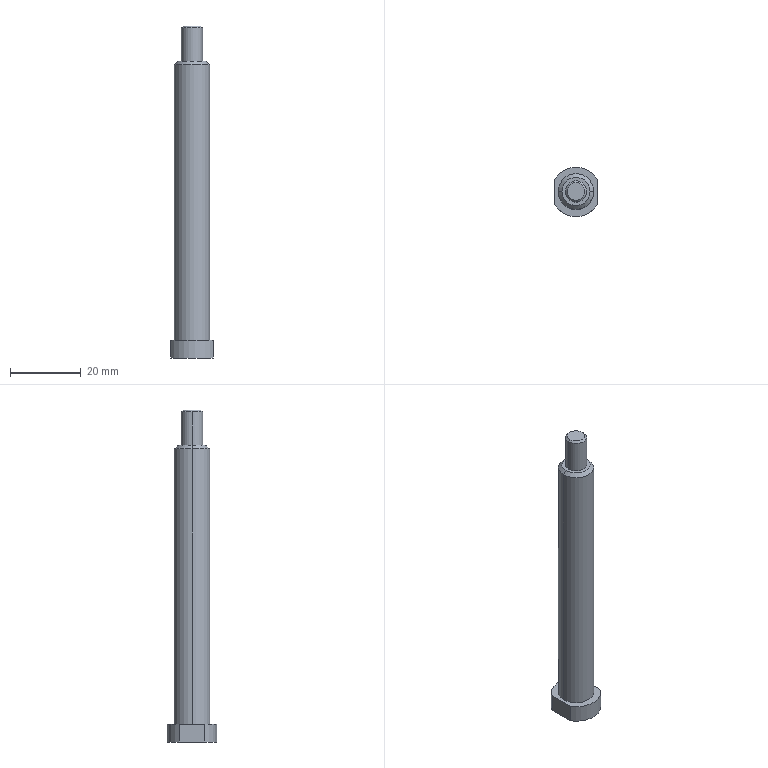Component | SolidWorks | ZTDJ-L-400-04-21-MaterialPortBagClamp-Axis5-2 | 1 solid | 16 faces | box 12 x 14 x 94 mm | volume 7191 mm3 | cylinder 6 | plane 6 | cone 4 | commonest cylinder face diameters 6 x2 10 x2 14 x2 | material 1023 Carbon Steel Sheet (SS)
STEP:
#1=COLOUR_RGB('',0.7922,0.8196,0.9333);
#2=FILL_AREA_STYLE_COLOUR('',#1);
#3=FILL_AREA_STYLE('',(#2));
#4=SURFACE_STYLE_FILL_AREA(#3);
#5=SURFACE_SIDE_STYLE('',(#4));
#6=SURFACE_STYLE_USAGE(.BOTH.,#5);
#7=PRESENTATION_STYLE_ASSIGNMENT((#6));
#8=CARTESIAN_POINT('',(-3.383,-3.314,13.346));
#9=VERTEX_POINT('',#8);
#10=CARTESIAN_POINT('',(-3.58,-3.314,13.346));
#11=VERTEX_POINT('',#10);
#12=CARTESIAN_POINT('',(-3.482,-3.314,13.346));
#13=DIRECTION('',(0.,0.,1.));
#14=DIRECTION('',(1.,0.,0.));
#15=AXIS2_PLACEMENT_3D('',#12,#13,#14);
#16=CIRCLE('',#15,0.09843);
#17=EDGE_CURVE('',#9,#11,#16,.T.);
#18=ORIENTED_EDGE('',*,*,#17,.F.);
#19=CARTESIAN_POINT('',(-3.364,-3.314,13.327));
#20=VERTEX_POINT('',#19);
#21=CARTESIAN_POINT('',(-3.383,-3.314,13.346));
#22=DIRECTION('',(0.7071,0.,-0.7071));
#23=VECTOR('',#22,39.37);
#24=LINE('',#21,#23);
#25=EDGE_CURVE('',#9,#20,#24,.T.);
#26=ORIENTED_EDGE('',*,*,#25,.T.);
#27=CARTESIAN_POINT('',(-3.6,-3.314,13.327));
#28=VERTEX_POINT('',#27);
#29=CARTESIAN_POINT('',(-3.482,-3.314,13.327));
#30=DIRECTION('',(0.,0.,-1.));
#31=DIRECTION('',(1.,0.,0.));
#32=AXIS2_PLACEMENT_3D('',#29,#30,#31);
#33=CIRCLE('',#32,0.1181);
#34=EDGE_CURVE('',#28,#20,#33,.T.);
#35=ORIENTED_EDGE('',*,*,#34,.F.);
#36=CARTESIAN_POINT('',(-3.58,-3.314,13.346));
#37=DIRECTION('',(-0.7071,0.,-0.7071));
#38=VECTOR('',#37,39.37);
#39=LINE('',#36,#38);
#40=EDGE_CURVE('',#11,#28,#39,.T.);
#41=ORIENTED_EDGE('',*,*,#40,.F.);
#42=EDGE_LOOP('',(#18,#26,#35,#41));
#43=FACE_OUTER_BOUND('',#42,.T.);
#44=CARTESIAN_POINT('',(-3.482,-3.314,13.346));
#45=DIRECTION('',(0.,0.,-1.));
#46=DIRECTION('',(-1.,0.,0.));
#47=AXIS2_PLACEMENT_3D('',#44,#45,#46);
#48=CONICAL_SURFACE('',#47,0.09843,0.7854);
#49=ADVANCED_FACE('',(#43),#48,.T.);
#50=ORIENTED_EDGE('',*,*,#34,.T.);
#51=CARTESIAN_POINT('',(-3.364,-3.314,12.953));
#52=VERTEX_POINT('',#51);
#53=CARTESIAN_POINT('',(-3.364,-3.314,13.346));
#54=DIRECTION('',(0.,0.,-1.));
#55=VECTOR('',#54,39.37);
#56=LINE('',#53,#55);
#57=EDGE_CURVE('',#20,#52,#56,.T.);
#58=ORIENTED_EDGE('',*,*,#57,.T.);
#59=CARTESIAN_POINT('',(-3.6,-3.314,12.953));
#60=VERTEX_POINT('',#59);
#61=CARTESIAN_POINT('',(-3.482,-3.314,12.953));
#62=DIRECTION('',(0.,0.,1.));
#63=DIRECTION('',(1.,0.,0.));
#64=AXIS2_PLACEMENT_3D('',#61,#62,#63);
#65=CIRCLE('',#64,0.1181);
#66=EDGE_CURVE('',#52,#60,#65,.T.);
#67=ORIENTED_EDGE('',*,*,#66,.T.);
#68=CARTESIAN_POINT('',(-3.6,-3.314,13.346));
#69=DIRECTION('',(0.,0.,-1.));
#70=VECTOR('',#69,39.37);
#71=LINE('',#68,#70);
#72=EDGE_CURVE('',#28,#60,#71,.T.);
#73=ORIENTED_EDGE('',*,*,#72,.F.);
#74=EDGE_LOOP('',(#50,#58,#67,#73));
#75=FACE_OUTER_BOUND('',#74,.T.);
#76=CARTESIAN_POINT('',(-3.482,-3.314,13.346));
#77=DIRECTION('',(0.,0.,-1.));
#78=DIRECTION('',(-1.,0.,0.));
#79=AXIS2_PLACEMENT_3D('',#76,#77,#78);
#80=CYLINDRICAL_SURFACE('',#79,0.1181);
#81=ADVANCED_FACE('',(#75),#80,.T.);
#82=CARTESIAN_POINT('',(-3.324,-3.314,12.953));
#83=VERTEX_POINT('',#82);
#84=CARTESIAN_POINT('',(-3.639,-3.314,12.953));
#85=VERTEX_POINT('',#84);
#86=CARTESIAN_POINT('',(-3.482,-3.314,12.953));
#87=DIRECTION('',(0.,0.,1.));
#88=DIRECTION('',(1.,0.,0.));
#89=AXIS2_PLACEMENT_3D('',#86,#87,#88);
#90=CIRCLE('',#89,0.1575);
#91=EDGE_CURVE('',#83,#85,#90,.T.);
#92=ORIENTED_EDGE('',*,*,#91,.F.);
#93=CARTESIAN_POINT('',(-3.285,-3.314,12.913));
#94=VERTEX_POINT('',#93);
#95=CARTESIAN_POINT('',(-3.324,-3.314,12.953));
#96=DIRECTION('',(0.7071,0.,-0.7071));
#97=VECTOR('',#96,39.37);
#98=LINE('',#95,#97);
#99=EDGE_CURVE('',#83,#94,#98,.T.);
#100=ORIENTED_EDGE('',*,*,#99,.T.);
#101=CARTESIAN_POINT('',(-3.679,-3.314,12.913));
#102=VERTEX_POINT('',#101);
#103=CARTESIAN_POINT('',(-3.482,-3.314,12.913));
#104=DIRECTION('',(0.,0.,-1.));
#105=DIRECTION('',(1.,0.,0.));
#106=AXIS2_PLACEMENT_3D('',#103,#104,#105);
#107=CIRCLE('',#106,0.1969);
#108=EDGE_CURVE('',#102,#94,#107,.T.);
#109=ORIENTED_EDGE('',*,*,#108,.F.);
#110=CARTESIAN_POINT('',(-3.639,-3.314,12.953));
#111=DIRECTION('',(-0.7071,0.,-0.7071));
#112=VECTOR('',#111,39.37);
#113=LINE('',#110,#112);
#114=EDGE_CURVE('',#85,#102,#113,.T.);
#115=ORIENTED_EDGE('',*,*,#114,.F.);
#116=EDGE_LOOP('',(#92,#100,#109,#115));
#117=FACE_OUTER_BOUND('',#116,.T.);
#118=CARTESIAN_POINT('',(-3.482,-3.314,12.953));
#119=DIRECTION('',(0.,0.,-1.));
#120=DIRECTION('',(-1.,0.,0.));
#121=AXIS2_PLACEMENT_3D('',#118,#119,#120);
#122=CONICAL_SURFACE('',#121,0.1575,0.7854);
#123=ADVANCED_FACE('',(#117),#122,.T.);
#124=ORIENTED_EDGE('',*,*,#108,.T.);
#125=CARTESIAN_POINT('',(-3.285,-3.314,9.843));
#126=VERTEX_POINT('',#125);
#127=CARTESIAN_POINT('',(-3.285,-3.314,12.953));
#128=DIRECTION('',(0.,0.,-1.));
#129=VECTOR('',#128,39.37);
#130=LINE('',#127,#129);
#131=EDGE_CURVE('',#94,#126,#130,.T.);
#132=ORIENTED_EDGE('',*,*,#131,.T.);
#133=CARTESIAN_POINT('',(-3.679,-3.314,9.843));
#134=VERTEX_POINT('',#133);
#135=CARTESIAN_POINT('',(-3.482,-3.314,9.843));
#136=DIRECTION('',(0.,0.,-1.));
#137=DIRECTION('',(-1.,0.,0.));
#138=AXIS2_PLACEMENT_3D('',#135,#136,#137);
#139=CIRCLE('',#138,0.1969);
#140=EDGE_CURVE('',#134,#126,#139,.T.);
#141=ORIENTED_EDGE('',*,*,#140,.F.);
#142=CARTESIAN_POINT('',(-3.679,-3.314,12.953));
#143=DIRECTION('',(0.,0.,-1.));
#144=VECTOR('',#143,39.37);
#145=LINE('',#142,#144);
#146=EDGE_CURVE('',#102,#134,#145,.T.);
#147=ORIENTED_EDGE('',*,*,#146,.F.);
#148=EDGE_LOOP('',(#124,#132,#141,#147));
#149=FACE_OUTER_BOUND('',#148,.T.);
#150=CARTESIAN_POINT('',(-3.482,-3.314,12.953));
#151=DIRECTION('',(0.,0.,-1.));
#152=DIRECTION('',(-1.,0.,0.));
#153=AXIS2_PLACEMENT_3D('',#150,#151,#152);
#154=CYLINDRICAL_SURFACE('',#153,0.1969);
#155=ADVANCED_FACE('',(#149),#154,.T.);
#156=CARTESIAN_POINT('',(-3.246,-3.456,9.646));
#157=VERTEX_POINT('',#156);
#158=CARTESIAN_POINT('',(-3.718,-3.456,9.646));
#159=VERTEX_POINT('',#158);
#160=CARTESIAN_POINT('',(-3.482,-3.314,9.646));
#161=DIRECTION('',(0.,0.,-1.));
#162=DIRECTION('',(-1.,0.,0.));
#163=AXIS2_PLACEMENT_3D('',#160,#161,#162);
#164=CIRCLE('',#163,0.2756);
#165=EDGE_CURVE('',#157,#159,#164,.T.);
#166=ORIENTED_EDGE('',*,*,#165,.F.);
#167=CARTESIAN_POINT('',(-3.246,-3.456,9.843));
#168=VERTEX_POINT('',#167);
#169=CARTESIAN_POINT('',(-3.246,-3.456,9.449));
#170=DIRECTION('',(0.,0.,1.));
#171=VECTOR('',#170,39.37);
#172=LINE('',#169,#171);
#173=EDGE_CURVE('',#157,#168,#172,.T.);
#174=ORIENTED_EDGE('',*,*,#173,.T.);
#175=CARTESIAN_POINT('',(-3.718,-3.456,9.843));
#176=VERTEX_POINT('',#175);
#177=CARTESIAN_POINT('',(-3.482,-3.314,9.843));
#178=DIRECTION('',(0.,0.,-1.));
#179=DIRECTION('',(-1.,0.,0.));
#180=AXIS2_PLACEMENT_3D('',#177,#178,#179);
#181=CIRCLE('',#180,0.2756);
#182=EDGE_CURVE('',#168,#176,#181,.T.);
#183=ORIENTED_EDGE('',*,*,#182,.T.);
#184=CARTESIAN_POINT('',(-3.718,-3.456,9.449));
#185=DIRECTION('',(0.,0.,1.));
#186=VECTOR('',#185,39.37);
#187=LINE('',#184,#186);
#188=EDGE_CURVE('',#159,#176,#187,.T.);
#189=ORIENTED_EDGE('',*,*,#188,.F.);
#190=EDGE_LOOP('',(#166,#174,#183,#189));
#191=FACE_OUTER_BOUND('',#190,.T.);
#192=CARTESIAN_POINT('',(-3.482,-3.314,9.646));
#193=DIRECTION('',(0.,0.,1.));
#194=DIRECTION('',(1.,0.,0.));
#195=AXIS2_PLACEMENT_3D('',#192,#193,#194);
#196=CYLINDRICAL_SURFACE('',#195,0.2756);
#197=ADVANCED_FACE('',(#191),#196,.T.);
#198=ORIENTED_EDGE('',*,*,#140,.T.);
#199=CARTESIAN_POINT('',(-3.482,-3.314,9.843));
#200=DIRECTION('',(0.,0.,-1.));
#201=DIRECTION('',(-1.,0.,0.));
#202=AXIS2_PLACEMENT_3D('',#199,#200,#201);
#203=CIRCLE('',#202,0.1969);
#204=EDGE_CURVE('',#126,#134,#203,.T.);
#205=ORIENTED_EDGE('',*,*,#204,.T.);
#206=EDGE_LOOP('',(#198,#205));
#207=FACE_BOUND('',#206,.T.);
#208=ORIENTED_EDGE('',*,*,#182,.F.);
#209=CARTESIAN_POINT('',(-3.246,-3.172,9.843));
#210=VERTEX_POINT('',#209);
#211=CARTESIAN_POINT('',(-3.246,-3.314,9.843));
#212=DIRECTION('',(0.,-1.,0.));
#213=VECTOR('',#212,39.37);
#214=LINE('',#211,#213);
#215=EDGE_CURVE('',#210,#168,#214,.T.);
#216=ORIENTED_EDGE('',*,*,#215,.F.);
#217=CARTESIAN_POINT('',(-3.718,-3.172,9.843));
#218=VERTEX_POINT('',#217);
#219=CARTESIAN_POINT('',(-3.482,-3.314,9.843));
#220=DIRECTION('',(0.,0.,-1.));
#221=DIRECTION('',(-1.,0.,0.));
#222=AXIS2_PLACEMENT_3D('',#219,#220,#221);
#223=CIRCLE('',#222,0.2756);
#224=EDGE_CURVE('',#218,#210,#223,.T.);
#225=ORIENTED_EDGE('',*,*,#224,.F.);
#226=CARTESIAN_POINT('',(-3.718,-3.314,9.843));
#227=DIRECTION('',(0.,-1.,0.));
#228=VECTOR('',#227,39.37);
#229=LINE('',#226,#228);
#230=EDGE_CURVE('',#218,#176,#229,.T.);
#231=ORIENTED_EDGE('',*,*,#230,.T.);
#232=EDGE_LOOP('',(#208,#216,#225,#231));
#233=FACE_OUTER_BOUND('',#232,.T.);
#234=CARTESIAN_POINT('',(-3.482,-3.314,9.843));
#235=DIRECTION('',(0.,0.,-1.));
#236=DIRECTION('',(-1.,0.,0.));
#237=AXIS2_PLACEMENT_3D('',#234,#235,#236);
#238=PLANE('',#237);
#239=ADVANCED_FACE('',(#207,#233),#238,.F.);
#240=ORIENTED_EDGE('',*,*,#224,.T.);
#241=CARTESIAN_POINT('',(-3.246,-3.172,9.646));
#242=VERTEX_POINT('',#241);
#243=CARTESIAN_POINT('',(-3.246,-3.172,9.449));
#244=DIRECTION('',(0.,0.,1.));
#245=VECTOR('',#244,39.37);
#246=LINE('',#243,#245);
#247=EDGE_CURVE('',#242,#210,#246,.T.);
#248=ORIENTED_EDGE('',*,*,#247,.F.);
#249=CARTESIAN_POINT('',(-3.718,-3.172,9.646));
#250=VERTEX_POINT('',#249);
#251=CARTESIAN_POINT('',(-3.482,-3.314,9.646));
#252=DIRECTION('',(0.,0.,-1.));
#253=DIRECTION('',(-1.,0.,0.));
#254=AXIS2_PLACEMENT_3D('',#251,#252,#253);
#255=CIRCLE('',#254,0.2756);
#256=EDGE_CURVE('',#250,#242,#255,.T.);
#257=ORIENTED_EDGE('',*,*,#256,.F.);
#258=CARTESIAN_POINT('',(-3.718,-3.172,9.449));
#259=DIRECTION('',(0.,0.,1.));
#260=VECTOR('',#259,39.37);
#261=LINE('',#258,#260);
#262=EDGE_CURVE('',#250,#218,#261,.T.);
#263=ORIENTED_EDGE('',*,*,#262,.T.);
#264=EDGE_LOOP('',(#240,#248,#257,#263));
#265=FACE_OUTER_BOUND('',#264,.T.);
#266=CARTESIAN_POINT('',(-3.482,-3.314,9.646));
#267=DIRECTION('',(0.,0.,1.));
#268=DIRECTION('',(1.,0.,0.));
#269=AXIS2_PLACEMENT_3D('',#266,#267,#268);
#270=CYLINDRICAL_SURFACE('',#269,0.2756);
#271=ADVANCED_FACE('',(#265),#270,.T.);
#272=CARTESIAN_POINT('',(-3.246,-3.314,9.646));
#273=DIRECTION('',(0.,1.,0.));
#274=VECTOR('',#273,39.37);
#275=LINE('',#272,#274);
#276=EDGE_CURVE('',#157,#242,#275,.T.);
#277=ORIENTED_EDGE('',*,*,#276,.F.);
#278=ORIENTED_EDGE('',*,*,#165,.T.);
#279=CARTESIAN_POINT('',(-3.718,-3.314,9.646));
#280=DIRECTION('',(0.,1.,0.));
#281=VECTOR('',#280,39.37);
#282=LINE('',#279,#281);
#283=EDGE_CURVE('',#159,#250,#282,.T.);
#284=ORIENTED_EDGE('',*,*,#283,.T.);
#285=ORIENTED_EDGE('',*,*,#256,.T.);
#286=EDGE_LOOP('',(#277,#278,#284,#285));
#287=FACE_OUTER_BOUND('',#286,.T.);
#288=CARTESIAN_POINT('',(-3.482,-3.314,9.646));
#289=DIRECTION('',(0.,0.,-1.));
#290=DIRECTION('',(-1.,0.,0.));
#291=AXIS2_PLACEMENT_3D('',#288,#289,#290);
#292=PLANE('',#291);
#293=ADVANCED_FACE('',(#287),#292,.T.);
#294=CARTESIAN_POINT('',(-3.482,-3.314,12.953));
#295=DIRECTION('',(0.,0.,1.));
#296=DIRECTION('',(1.,0.,0.));
#297=AXIS2_PLACEMENT_3D('',#294,#295,#296);
#298=CIRCLE('',#297,0.1575);
#299=EDGE_CURVE('',#85,#83,#298,.T.);
#300=ORIENTED_EDGE('',*,*,#299,.T.);
#301=ORIENTED_EDGE('',*,*,#91,.T.);
#302=EDGE_LOOP('',(#300,#301));
#303=FACE_OUTER_BOUND('',#302,.T.);
#304=CARTESIAN_POINT('',(-3.482,-3.314,12.953));
#305=DIRECTION('',(0.,0.,1.));
#306=DIRECTION('',(1.,0.,0.));
#307=AXIS2_PLACEMENT_3D('',#304,#305,#306);
#308=CIRCLE('',#307,0.1181);
#309=EDGE_CURVE('',#60,#52,#308,.T.);
#310=ORIENTED_EDGE('',*,*,#309,.F.);
#311=ORIENTED_EDGE('',*,*,#66,.F.);
#312=EDGE_LOOP('',(#310,#311));
#313=FACE_BOUND('',#312,.T.);
#314=CARTESIAN_POINT('',(-3.482,-3.314,12.953));
#315=DIRECTION('',(0.,0.,1.));
#316=DIRECTION('',(1.,0.,0.));
#317=AXIS2_PLACEMENT_3D('',#314,#315,#316);
#318=PLANE('',#317);
#319=ADVANCED_FACE('',(#303,#313),#318,.T.);
#320=ORIENTED_EDGE('',*,*,#131,.F.);
#321=CARTESIAN_POINT('',(-3.482,-3.314,12.913));
#322=DIRECTION('',(0.,0.,-1.));
#323=DIRECTION('',(1.,0.,0.));
#324=AXIS2_PLACEMENT_3D('',#321,#322,#323);
#325=CIRCLE('',#324,0.1969);
#326=EDGE_CURVE('',#94,#102,#325,.T.);
#327=ORIENTED_EDGE('',*,*,#326,.T.);
#328=ORIENTED_EDGE('',*,*,#146,.T.);
#329=ORIENTED_EDGE('',*,*,#204,.F.);
#330=EDGE_LOOP('',(#320,#327,#328,#329));
#331=FACE_OUTER_BOUND('',#330,.T.);
#332=CARTESIAN_POINT('',(-3.482,-3.314,12.953));
#333=DIRECTION('',(0.,0.,-1.));
#334=DIRECTION('',(-1.,0.,0.));
#335=AXIS2_PLACEMENT_3D('',#332,#333,#334);
#336=CYLINDRICAL_SURFACE('',#335,0.1969);
#337=ADVANCED_FACE('',(#331),#336,.T.);
#338=ORIENTED_EDGE('',*,*,#99,.F.);
#339=ORIENTED_EDGE('',*,*,#299,.F.);
#340=ORIENTED_EDGE('',*,*,#114,.T.);
#341=ORIENTED_EDGE('',*,*,#326,.F.);
#342=EDGE_LOOP('',(#338,#339,#340,#341));
#343=FACE_OUTER_BOUND('',#342,.T.);
#344=CARTESIAN_POINT('',(-3.482,-3.314,12.953));
#345=DIRECTION('',(0.,0.,-1.));
#346=DIRECTION('',(-1.,0.,0.));
#347=AXIS2_PLACEMENT_3D('',#344,#345,#346);
#348=CONICAL_SURFACE('',#347,0.1575,0.7854);
#349=ADVANCED_FACE('',(#343),#348,.T.);
#350=ORIENTED_EDGE('',*,*,#57,.F.);
#351=CARTESIAN_POINT('',(-3.482,-3.314,13.327));
#352=DIRECTION('',(0.,0.,-1.));
#353=DIRECTION('',(1.,0.,0.));
#354=AXIS2_PLACEMENT_3D('',#351,#352,#353);
#355=CIRCLE('',#354,0.1181);
#356=EDGE_CURVE('',#20,#28,#355,.T.);
#357=ORIENTED_EDGE('',*,*,#356,.T.);
#358=ORIENTED_EDGE('',*,*,#72,.T.);
#359=ORIENTED_EDGE('',*,*,#309,.T.);
#360=EDGE_LOOP('',(#350,#357,#358,#359));
#361=FACE_OUTER_BOUND('',#360,.T.);
#362=CARTESIAN_POINT('',(-3.482,-3.314,13.346));
#363=DIRECTION('',(0.,0.,-1.));
#364=DIRECTION('',(-1.,0.,0.));
#365=AXIS2_PLACEMENT_3D('',#362,#363,#364);
#366=CYLINDRICAL_SURFACE('',#365,0.1181);
#367=ADVANCED_FACE('',(#361),#366,.T.);
#368=CARTESIAN_POINT('',(-3.482,-3.314,13.346));
#369=DIRECTION('',(0.,0.,1.));
#370=DIRECTION('',(1.,0.,0.));
#371=AXIS2_PLACEMENT_3D('',#368,#369,#370);
#372=CIRCLE('',#371,0.09843);
#373=EDGE_CURVE('',#11,#9,#372,.T.);
#374=ORIENTED_EDGE('',*,*,#373,.T.);
#375=ORIENTED_EDGE('',*,*,#17,.T.);
#376=EDGE_LOOP('',(#374,#375));
#377=FACE_OUTER_BOUND('',#376,.T.);
#378=CARTESIAN_POINT('',(-3.482,-3.314,13.346));
#379=DIRECTION('',(0.,0.,1.));
#380=DIRECTION('',(1.,0.,0.));
#381=AXIS2_PLACEMENT_3D('',#378,#379,#380);
#382=PLANE('',#381);
#383=ADVANCED_FACE('',(#377),#382,.T.);
#384=ORIENTED_EDGE('',*,*,#25,.F.);
#385=ORIENTED_EDGE('',*,*,#373,.F.);
#386=ORIENTED_EDGE('',*,*,#40,.T.);
#387=ORIENTED_EDGE('',*,*,#356,.F.);
#388=EDGE_LOOP('',(#384,#385,#386,#387));
#389=FACE_OUTER_BOUND('',#388,.T.);
#390=CARTESIAN_POINT('',(-3.482,-3.314,13.346));
#391=DIRECTION('',(0.,0.,-1.));
#392=DIRECTION('',(-1.,0.,0.));
#393=AXIS2_PLACEMENT_3D('',#390,#391,#392);
#394=CONICAL_SURFACE('',#393,0.09843,0.7854);
#395=ADVANCED_FACE('',(#389),#394,.T.);
#396=ORIENTED_EDGE('',*,*,#188,.T.);
#397=ORIENTED_EDGE('',*,*,#230,.F.);
#398=ORIENTED_EDGE('',*,*,#262,.F.);
#399=ORIENTED_EDGE('',*,*,#283,.F.);
#400=EDGE_LOOP('',(#396,#397,#398,#399));
#401=FACE_OUTER_BOUND('',#400,.T.);
#402=CARTESIAN_POINT('',(-3.718,-3.314,9.449));
#403=DIRECTION('',(-1.,0.,0.));
#404=DIRECTION('',(0.,0.,1.));
#405=AXIS2_PLACEMENT_3D('',#402,#403,#404);
#406=PLANE('',#405);
#407=ADVANCED_FACE('',(#401),#406,.T.);
#408=ORIENTED_EDGE('',*,*,#276,.T.);
#409=ORIENTED_EDGE('',*,*,#247,.T.);
#410=ORIENTED_EDGE('',*,*,#215,.T.);
#411=ORIENTED_EDGE('',*,*,#173,.F.);
#412=EDGE_LOOP('',(#408,#409,#410,#411));
#413=FACE_OUTER_BOUND('',#412,.T.);
#414=CARTESIAN_POINT('',(-3.246,-3.314,9.449));
#415=DIRECTION('',(-1.,0.,0.));
#416=DIRECTION('',(0.,0.,1.));
#417=AXIS2_PLACEMENT_3D('',#414,#415,#416);
#418=PLANE('',#417);
#419=ADVANCED_FACE('',(#413),#418,.F.);
#420=CLOSED_SHELL('',(#49,#81,#123,#155,#197,#239,#271,#293,#319,#337,#349,#367,#383,#395,#407,#419));
#421=MANIFOLD_SOLID_BREP('',#420);
#422=STYLED_ITEM('',(#7),#421);
#423=(LENGTH_UNIT()NAMED_UNIT(*)SI_UNIT($,.METRE.));
#424=LENGTH_MEASURE_WITH_UNIT(LENGTH_MEASURE(0.0254),#423);
#425=DIMENSIONAL_EXPONENTS(1.,0.,0.,0.,0.,0.,0.);
#426=(CONVERSION_BASED_UNIT('',#424)LENGTH_UNIT()NAMED_UNIT(#425));
#427=UNCERTAINTY_MEASURE_WITH_UNIT(LENGTH_MEASURE(0.00001),#426,'','');
#428=(NAMED_UNIT(*)PLANE_ANGLE_UNIT()SI_UNIT($,.RADIAN.));
#429=(NAMED_UNIT(*)SI_UNIT($,.STERADIAN.)SOLID_ANGLE_UNIT());
#430=(GEOMETRIC_REPRESENTATION_CONTEXT(3)GLOBAL_UNCERTAINTY_ASSIGNED_CONTEXT((#427))GLOBAL_UNIT_ASSIGNED_CONTEXT((#426,#428,#429))REPRESENTATION_CONTEXT('',''));
#431=MECHANICAL_DESIGN_GEOMETRIC_PRESENTATION_REPRESENTATION('',(#422),#430);
#432=CARTESIAN_POINT('',(0.,0.,0.));
#433=DIRECTION('',(0.,0.,1.));
#434=DIRECTION('',(1.,0.,0.));
#435=AXIS2_PLACEMENT_3D('',#432,#433,#434);
#436=(LENGTH_UNIT()NAMED_UNIT(*)SI_UNIT($,.METRE.));
#437=LENGTH_MEASURE_WITH_UNIT(LENGTH_MEASURE(0.0254),#436);
#438=DIMENSIONAL_EXPONENTS(1.,0.,0.,0.,0.,0.,0.);
#439=(CONVERSION_BASED_UNIT('',#437)LENGTH_UNIT()NAMED_UNIT(#438));
#440=UNCERTAINTY_MEASURE_WITH_UNIT(LENGTH_MEASURE(0.00001),#439,'','');
#441=(NAMED_UNIT(*)PLANE_ANGLE_UNIT()SI_UNIT($,.RADIAN.));
#442=(NAMED_UNIT(*)SI_UNIT($,.STERADIAN.)SOLID_ANGLE_UNIT());
#443=(GEOMETRIC_REPRESENTATION_CONTEXT(3)GLOBAL_UNCERTAINTY_ASSIGNED_CONTEXT((#440))GLOBAL_UNIT_ASSIGNED_CONTEXT((#439,#441,#442))REPRESENTATION_CONTEXT('',''));
#444=ADVANCED_BREP_SHAPE_REPRESENTATION('',(#421,#435),#443);
#445=PRESENTATION_LAYER_ASSIGNMENT('','',(#422));